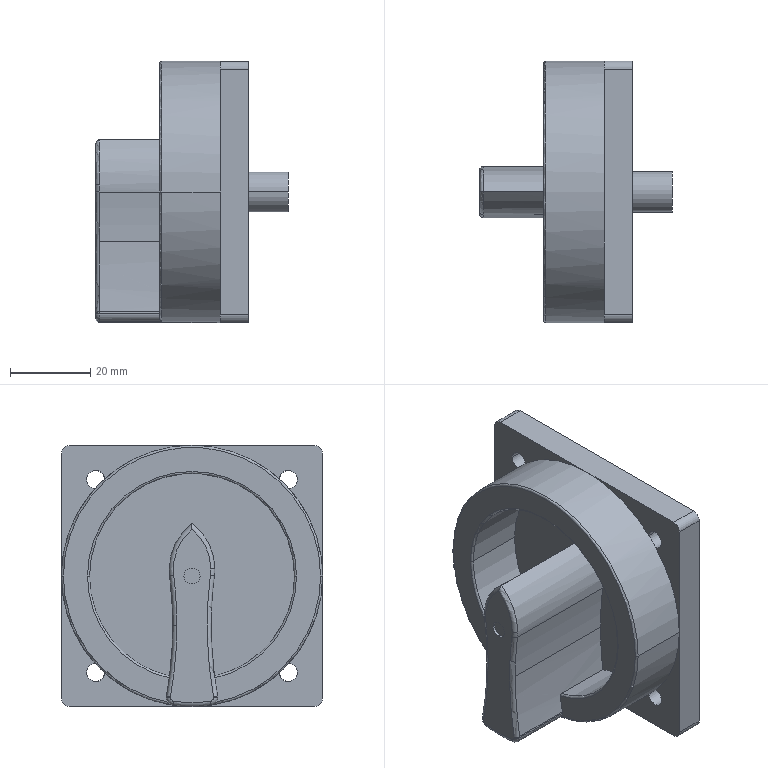Component | SolidWorks | PowerSwitchTDS25-FRR-1 | 1 solid | 65 faces | volume 61605 mm3 | cylinder 30 | plane 18 | torus 17 | commonest cylinder face diameters 4 x9 4.5 x8 51 x3 195.952 x3 28 x3 10 x2 65 x2